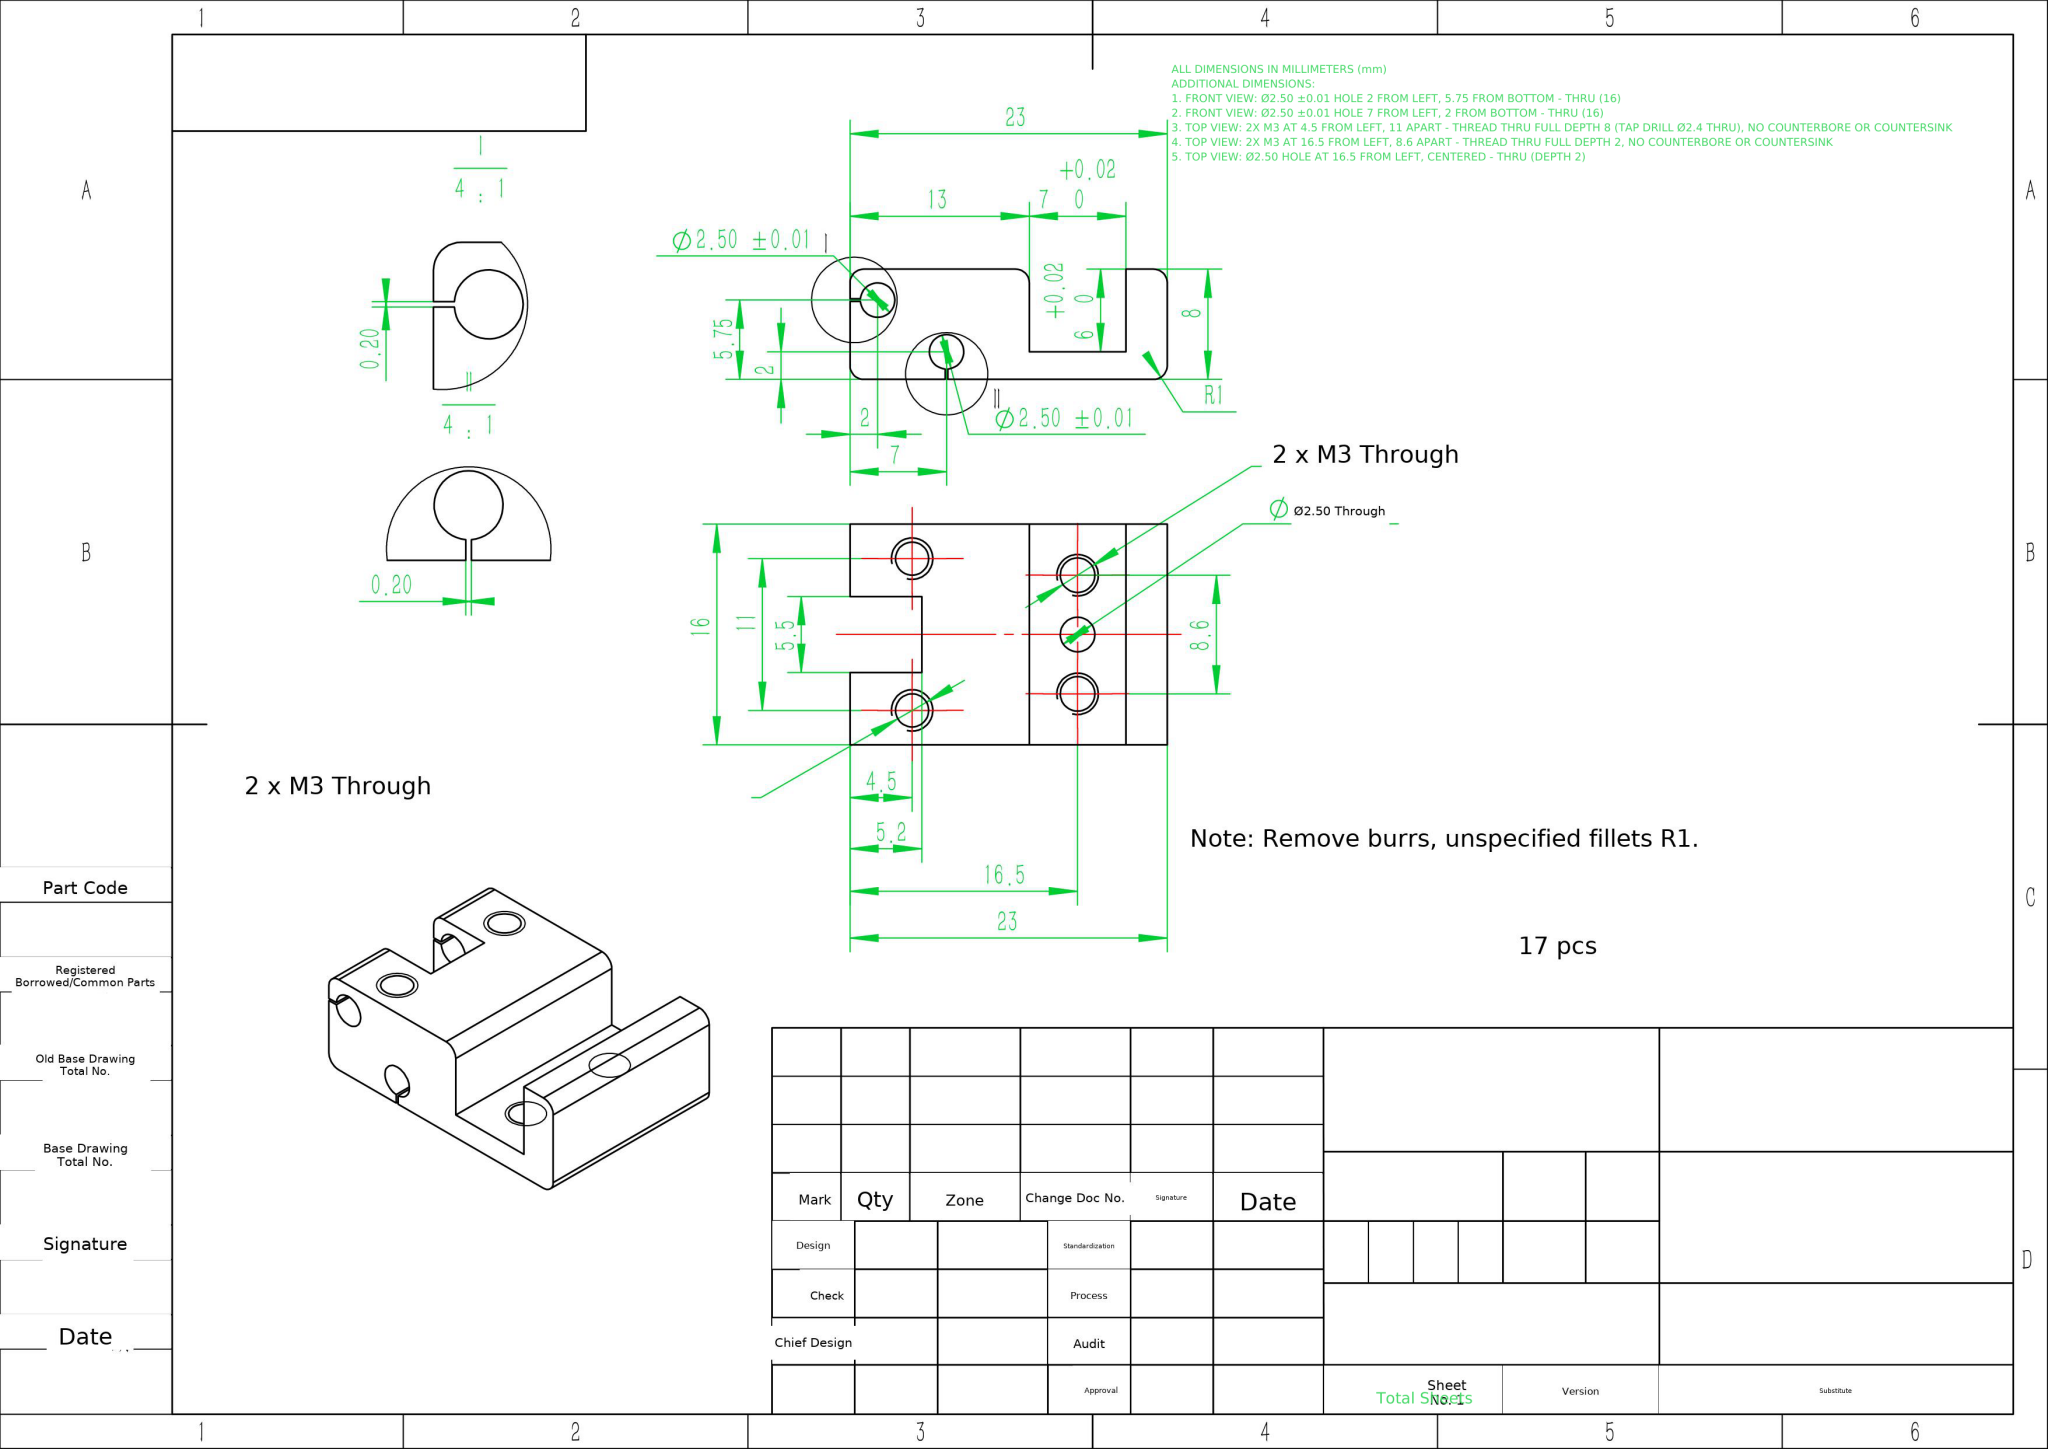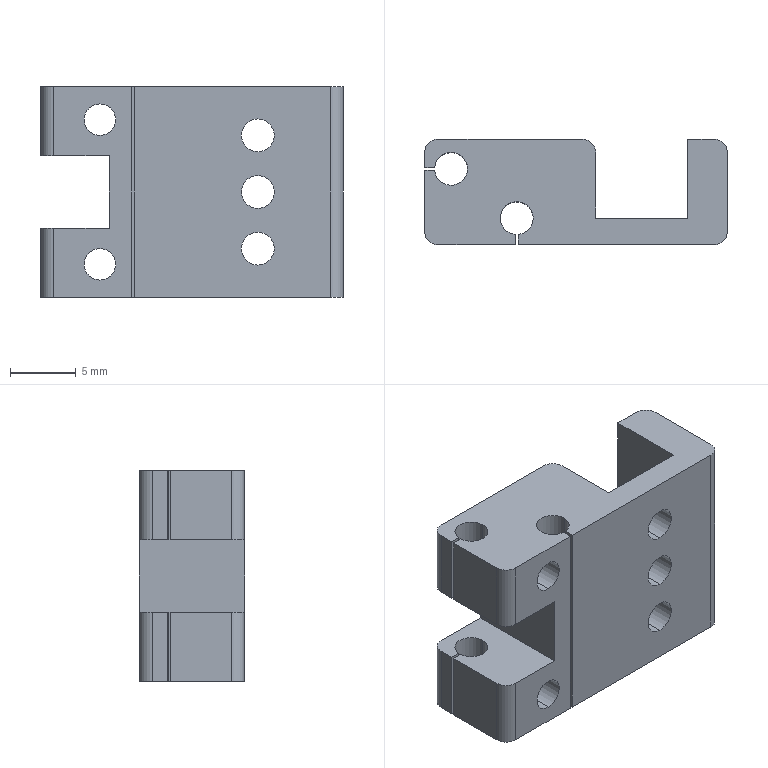Part | NX | mm | 1 solid | 47 faces | box 23 x 8 x 16 mm | volume 1792 mm3 | cylinder 24 | plane 23 | commonest cylinder face diameters 2.5 x13 2 x7 2.4 x4